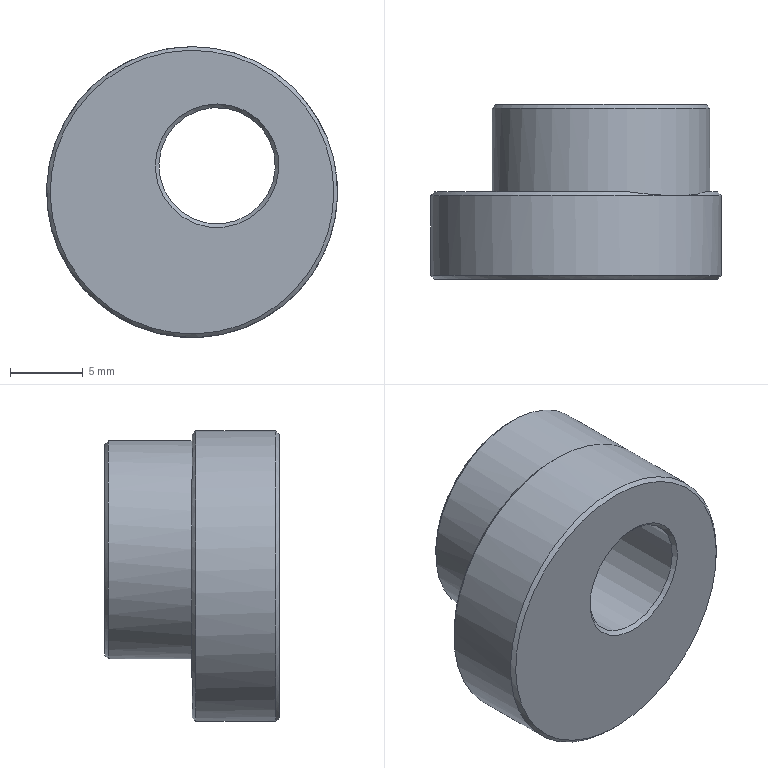Component | NX | ECCENTRIC_WHEEL | 1 solid | 11 faces | box 20 x 12 x 20 mm | volume 2335 mm3 | cone 5 | plane 3 | cylinder 3 | commonest cylinder face diameters 20 x1 15 x1 8 x1
STEP:
#1=CARTESIAN_POINT('',(0.,0.,0.));
#2=DIRECTION('',(0.,0.,1.));
#3=DIRECTION('',(1.,0.,0.));
#4=AXIS2_PLACEMENT_3D('',#1,#2,#3);
#5=CARTESIAN_POINT('',(7.185,-7.75,43.152));
#6=VERTEX_POINT('',#5);
#7=CARTESIAN_POINT('',(1.796,-7.75,48.282));
#8=VERTEX_POINT('',#7);
#9=CARTESIAN_POINT('',(-0.,-7.75,41.));
#10=DIRECTION('',(0.,1.,0.));
#11=DIRECTION('',(-0.7243,0.,0.6895));
#12=AXIS2_PLACEMENT_3D('',#9,#10,#11);
#13=CIRCLE('',#12,7.5);
#14=CARTESIAN_POINT('',(-1.724,-7.75,39.189));
#15=DIRECTION('',(0.,1.,0.));
#16=DIRECTION('',(-0.7243,0.,0.6895));
#17=AXIS2_PLACEMENT_3D('',#14,#15,#16);
#18=PLANE('',#17);
#19=CARTESIAN_POINT('',(0.,2.5));
#20=DIRECTION('',(1.,0.));
#21=AXIS2_PLACEMENT_2D('',#19,#20);
#22=CIRCLE('',#21,7.5);
#23=(GEOMETRIC_REPRESENTATION_CONTEXT(2)PARAMETRIC_REPRESENTATION_CONTEXT()REPRESENTATION_CONTEXT('',''));
#24=DEFINITIONAL_REPRESENTATION('',(#22),#23);
#25=PCURVE('',#18,#24);
#26=CARTESIAN_POINT('',(-0.,-1.75,41.));
#27=DIRECTION('',(0.,-1.,0.));
#28=DIRECTION('',(0.7243,0.,-0.6895));
#29=AXIS2_PLACEMENT_3D('',#26,#27,#28);
#30=CYLINDRICAL_SURFACE('',#29,7.5);
#31=CARTESIAN_POINT('',(9.425,6.));
#32=DIRECTION('',(-1.,0.));
#33=VECTOR('',#32,1.);
#34=LINE('',#31,#33);
#35=(GEOMETRIC_REPRESENTATION_CONTEXT(2)PARAMETRIC_REPRESENTATION_CONTEXT()REPRESENTATION_CONTEXT('',''));
#36=DEFINITIONAL_REPRESENTATION('',(#34),#35);
#37=PCURVE('',#30,#36);
#38=SURFACE_CURVE('',#13,(#25,#37),.PCURVE_S1.);
#39=EDGE_CURVE('',#6,#8,#38,.T.);
#40=ORIENTED_EDGE('',*,*,#39,.F.);
#41=CARTESIAN_POINT('',(-1.724,-7.75,39.189));
#42=DIRECTION('',(0.,1.,0.));
#43=DIRECTION('',(-0.7243,0.,0.6895));
#44=AXIS2_PLACEMENT_3D('',#41,#42,#43);
#45=CIRCLE('',#44,9.75);
#46=CARTESIAN_POINT('',(0.,0.));
#47=DIRECTION('',(1.,0.));
#48=AXIS2_PLACEMENT_2D('',#46,#47);
#49=CIRCLE('',#48,9.75);
#50=(GEOMETRIC_REPRESENTATION_CONTEXT(2)PARAMETRIC_REPRESENTATION_CONTEXT()REPRESENTATION_CONTEXT('',''));
#51=DEFINITIONAL_REPRESENTATION('',(#49),#50);
#52=PCURVE('',#18,#51);
#53=CARTESIAN_POINT('',(-1.724,-8.,39.189));
#54=DIRECTION('',(0.,-1.,0.));
#55=DIRECTION('',(0.7243,0.,-0.6895));
#56=AXIS2_PLACEMENT_3D('',#53,#54,#55);
#57=CONICAL_SURFACE('',#56,10.,0.7854);
#58=CARTESIAN_POINT('',(9.425,-0.25));
#59=DIRECTION('',(-1.,0.));
#60=VECTOR('',#59,1.);
#61=LINE('',#58,#60);
#62=(GEOMETRIC_REPRESENTATION_CONTEXT(2)PARAMETRIC_REPRESENTATION_CONTEXT()REPRESENTATION_CONTEXT('',''));
#63=DEFINITIONAL_REPRESENTATION('',(#61),#62);
#64=PCURVE('',#57,#63);
#65=SURFACE_CURVE('',#45,(#52,#64),.PCURVE_S1.);
#66=EDGE_CURVE('',#6,#8,#65,.T.);
#67=ORIENTED_EDGE('',*,*,#66,.T.);
#68=EDGE_LOOP('',(#40,#67));
#69=FACE_BOUND('',#68,.T.);
#70=ADVANCED_FACE('',(#69),#18,.T.);
#71=CARTESIAN_POINT('',(3.078,-13.75,38.07));
#72=VERTEX_POINT('',#71);
#73=CARTESIAN_POINT('',(-0.,-13.75,41.));
#74=DIRECTION('',(0.,1.,0.));
#75=DIRECTION('',(0.7243,0.,-0.6895));
#76=AXIS2_PLACEMENT_3D('',#73,#74,#75);
#77=CIRCLE('',#76,4.25);
#78=CARTESIAN_POINT('',(-1.724,-13.75,39.189));
#79=DIRECTION('',(0.,-1.,0.));
#80=DIRECTION('',(0.7243,0.,-0.6895));
#81=AXIS2_PLACEMENT_3D('',#78,#79,#80);
#82=PLANE('',#81);
#83=CARTESIAN_POINT('',(4.25,2.5));
#84=CARTESIAN_POINT('',(4.25,-4.861));
#85=CARTESIAN_POINT('',(-2.125,-1.181));
#86=CARTESIAN_POINT('',(-8.5,2.5));
#87=CARTESIAN_POINT('',(-2.125,6.181));
#88=CARTESIAN_POINT('',(4.25,9.861));
#89=CARTESIAN_POINT('',(4.25,2.5));
#90=(BOUNDED_CURVE()B_SPLINE_CURVE(2,(#83,#84,#85,#86,#87,#88,#89),.UNSPECIFIED.,.T.,.F.)B_SPLINE_CURVE_WITH_KNOTS((1,2,2,2,2,1),(-2.094,0.,2.094,4.189,6.283,8.378),.UNSPECIFIED.)CURVE()GEOMETRIC_REPRESENTATION_ITEM()RATIONAL_B_SPLINE_CURVE((1.,0.5,1.,0.5,1.,0.5,1.))REPRESENTATION_ITEM(''));
#91=(GEOMETRIC_REPRESENTATION_CONTEXT(2)PARAMETRIC_REPRESENTATION_CONTEXT()REPRESENTATION_CONTEXT('',''));
#92=DEFINITIONAL_REPRESENTATION('',(#90),#91);
#93=PCURVE('',#82,#92);
#94=CARTESIAN_POINT('',(-0.,-13.5,41.));
#95=DIRECTION('',(0.,-1.,0.));
#96=DIRECTION('',(0.7243,0.,-0.6895));
#97=AXIS2_PLACEMENT_3D('',#94,#95,#96);
#98=CONICAL_SURFACE('',#97,4.,0.7854);
#99=CARTESIAN_POINT('',(6.283,0.25));
#100=DIRECTION('',(-1.,-0.));
#101=VECTOR('',#100,1.);
#102=LINE('',#99,#101);
#103=(GEOMETRIC_REPRESENTATION_CONTEXT(2)PARAMETRIC_REPRESENTATION_CONTEXT()REPRESENTATION_CONTEXT('',''));
#104=DEFINITIONAL_REPRESENTATION('',(#102),#103);
#105=PCURVE('',#98,#104);
#106=SURFACE_CURVE('',#77,(#93,#105),.PCURVE_S1.);
#107=EDGE_CURVE('',#72,#72,#106,.T.);
#108=ORIENTED_EDGE('',*,*,#107,.T.);
#109=EDGE_LOOP('',(#108));
#110=FACE_BOUND('',#109,.T.);
#111=CARTESIAN_POINT('',(5.338,-13.75,32.467));
#112=VERTEX_POINT('',#111);
#113=CARTESIAN_POINT('',(-1.724,-13.75,39.189));
#114=DIRECTION('',(0.,-1.,0.));
#115=DIRECTION('',(0.7243,0.,-0.6895));
#116=AXIS2_PLACEMENT_3D('',#113,#114,#115);
#117=CIRCLE('',#116,9.75);
#118=CARTESIAN_POINT('',(0.,0.));
#119=DIRECTION('',(1.,0.));
#120=AXIS2_PLACEMENT_2D('',#118,#119);
#121=CIRCLE('',#120,9.75);
#122=(GEOMETRIC_REPRESENTATION_CONTEXT(2)PARAMETRIC_REPRESENTATION_CONTEXT()REPRESENTATION_CONTEXT('',''));
#123=DEFINITIONAL_REPRESENTATION('',(#121),#122);
#124=PCURVE('',#82,#123);
#125=CARTESIAN_POINT('',(-1.724,-13.5,39.189));
#126=DIRECTION('',(0.,1.,0.));
#127=DIRECTION('',(-0.7243,0.,0.6895));
#128=AXIS2_PLACEMENT_3D('',#125,#126,#127);
#129=CONICAL_SURFACE('',#128,10.,0.7854);
#130=CARTESIAN_POINT('',(9.425,-0.25));
#131=DIRECTION('',(-1.,0.));
#132=VECTOR('',#131,1.);
#133=LINE('',#130,#132);
#134=(GEOMETRIC_REPRESENTATION_CONTEXT(2)PARAMETRIC_REPRESENTATION_CONTEXT()REPRESENTATION_CONTEXT('',''));
#135=DEFINITIONAL_REPRESENTATION('',(#133),#134);
#136=PCURVE('',#129,#135);
#137=SURFACE_CURVE('',#117,(#124,#136),.PCURVE_S1.);
#138=EDGE_CURVE('',#112,#112,#137,.T.);
#139=ORIENTED_EDGE('',*,*,#138,.T.);
#140=EDGE_LOOP('',(#139));
#141=FACE_BOUND('',#140,.T.);
#142=ADVANCED_FACE('',(#110,#141),#82,.T.);
#143=CARTESIAN_POINT('',(5.519,-13.5,32.294));
#144=VERTEX_POINT('',#143);
#145=CARTESIAN_POINT('',(5.171,-13.5,46.432));
#146=VERTEX_POINT('',#145);
#147=CARTESIAN_POINT('',(-1.724,-13.5,39.189));
#148=DIRECTION('',(0.,1.,0.));
#149=DIRECTION('',(0.7243,0.,-0.6895));
#150=AXIS2_PLACEMENT_3D('',#147,#148,#149);
#151=CIRCLE('',#150,10.);
#152=CARTESIAN_POINT('',(-1.724,-13.75,39.189));
#153=DIRECTION('',(0.,1.,0.));
#154=DIRECTION('',(-0.7243,0.,0.6895));
#155=AXIS2_PLACEMENT_3D('',#152,#153,#154);
#156=CYLINDRICAL_SURFACE('',#155,10.);
#157=CARTESIAN_POINT('',(3.142,0.25));
#158=DIRECTION('',(1.,0.));
#159=VECTOR('',#158,1.);
#160=LINE('',#157,#159);
#161=(GEOMETRIC_REPRESENTATION_CONTEXT(2)PARAMETRIC_REPRESENTATION_CONTEXT()REPRESENTATION_CONTEXT('',''));
#162=DEFINITIONAL_REPRESENTATION('',(#160),#161);
#163=PCURVE('',#156,#162);
#164=CARTESIAN_POINT('',(3.142,0.));
#165=DIRECTION('',(1.,-0.));
#166=VECTOR('',#165,1.);
#167=LINE('',#164,#166);
#168=(GEOMETRIC_REPRESENTATION_CONTEXT(2)PARAMETRIC_REPRESENTATION_CONTEXT()REPRESENTATION_CONTEXT('',''));
#169=DEFINITIONAL_REPRESENTATION('',(#167),#168);
#170=PCURVE('',#129,#169);
#171=SURFACE_CURVE('',#151,(#163,#170),.PCURVE_S1.);
#172=EDGE_CURVE('',#144,#146,#171,.T.);
#173=ORIENTED_EDGE('',*,*,#172,.T.);
#174=CARTESIAN_POINT('',(5.171,-8.,46.432));
#175=VERTEX_POINT('',#174);
#176=CARTESIAN_POINT('',(5.171,-13.5,46.432));
#177=CARTESIAN_POINT('',(5.171,-8.,46.432));
#178=B_SPLINE_CURVE_WITH_KNOTS('',1,(#176,#177),.UNSPECIFIED.,.F.,.F.,(2,2),(0.25,5.75),.PIECEWISE_BEZIER_KNOTS.);
#179=CARTESIAN_POINT('',(7.854,0.));
#180=DIRECTION('',(0.,1.));
#181=VECTOR('',#180,1.);
#182=LINE('',#179,#181);
#183=(GEOMETRIC_REPRESENTATION_CONTEXT(2)PARAMETRIC_REPRESENTATION_CONTEXT()REPRESENTATION_CONTEXT('',''));
#184=DEFINITIONAL_REPRESENTATION('',(#182),#183);
#185=PCURVE('',#156,#184);
#186=CARTESIAN_POINT('',(1.571,0.));
#187=DIRECTION('',(0.,1.));
#188=VECTOR('',#187,1.);
#189=LINE('',#186,#188);
#190=(GEOMETRIC_REPRESENTATION_CONTEXT(2)PARAMETRIC_REPRESENTATION_CONTEXT()REPRESENTATION_CONTEXT('',''));
#191=DEFINITIONAL_REPRESENTATION('',(#189),#190);
#192=PCURVE('',#156,#191);
#193=SEAM_CURVE('',#178,(#185,#192),.PCURVE_S1.);
#194=EDGE_CURVE('',#146,#175,#193,.T.);
#195=ORIENTED_EDGE('',*,*,#194,.T.);
#196=CARTESIAN_POINT('',(-1.724,-8.,39.189));
#197=DIRECTION('',(0.,-1.,0.));
#198=DIRECTION('',(-0.7243,0.,0.6895));
#199=AXIS2_PLACEMENT_3D('',#196,#197,#198);
#200=CIRCLE('',#199,10.);
#201=CARTESIAN_POINT('',(12.566,5.75));
#202=DIRECTION('',(-1.,0.));
#203=VECTOR('',#202,1.);
#204=LINE('',#201,#203);
#205=(GEOMETRIC_REPRESENTATION_CONTEXT(2)PARAMETRIC_REPRESENTATION_CONTEXT()REPRESENTATION_CONTEXT('',''));
#206=DEFINITIONAL_REPRESENTATION('',(#204),#205);
#207=PCURVE('',#156,#206);
#208=CARTESIAN_POINT('',(-3.142,0.));
#209=DIRECTION('',(1.,0.));
#210=VECTOR('',#209,1.);
#211=LINE('',#208,#210);
#212=(GEOMETRIC_REPRESENTATION_CONTEXT(2)PARAMETRIC_REPRESENTATION_CONTEXT()REPRESENTATION_CONTEXT('',''));
#213=DEFINITIONAL_REPRESENTATION('',(#211),#212);
#214=PCURVE('',#57,#213);
#215=SURFACE_CURVE('',#200,(#207,#214),.PCURVE_S1.);
#216=EDGE_CURVE('',#175,#175,#215,.T.);
#217=ORIENTED_EDGE('',*,*,#216,.T.);
#218=ORIENTED_EDGE('',*,*,#194,.F.);
#219=CARTESIAN_POINT('',(-1.724,-13.5,39.189));
#220=DIRECTION('',(0.,1.,0.));
#221=DIRECTION('',(0.7243,0.,-0.6895));
#222=AXIS2_PLACEMENT_3D('',#219,#220,#221);
#223=CIRCLE('',#222,10.);
#224=CARTESIAN_POINT('',(-3.142,0.25));
#225=DIRECTION('',(1.,0.));
#226=VECTOR('',#225,1.);
#227=LINE('',#224,#226);
#228=(GEOMETRIC_REPRESENTATION_CONTEXT(2)PARAMETRIC_REPRESENTATION_CONTEXT()REPRESENTATION_CONTEXT('',''));
#229=DEFINITIONAL_REPRESENTATION('',(#227),#228);
#230=PCURVE('',#156,#229);
#231=CARTESIAN_POINT('',(3.142,-0.));
#232=DIRECTION('',(1.,0.));
#233=VECTOR('',#232,1.);
#234=LINE('',#231,#233);
#235=(GEOMETRIC_REPRESENTATION_CONTEXT(2)PARAMETRIC_REPRESENTATION_CONTEXT()REPRESENTATION_CONTEXT('',''));
#236=DEFINITIONAL_REPRESENTATION('',(#234),#235);
#237=PCURVE('',#129,#236);
#238=SURFACE_CURVE('',#223,(#230,#237),.PCURVE_S1.);
#239=EDGE_CURVE('',#146,#144,#238,.T.);
#240=ORIENTED_EDGE('',*,*,#239,.T.);
#241=EDGE_LOOP('',(#173,#195,#217,#218,#240));
#242=FACE_BOUND('',#241,.T.);
#243=ADVANCED_FACE('',(#242),#156,.T.);
#244=CARTESIAN_POINT('',(-5.432,-2.,46.171));
#245=VERTEX_POINT('',#244);
#246=CARTESIAN_POINT('',(7.185,-2.,43.152));
#247=VERTEX_POINT('',#246);
#248=CARTESIAN_POINT('',(-0.,-2.,41.));
#249=DIRECTION('',(0.,-1.,0.));
#250=DIRECTION('',(-0.7243,0.,0.6895));
#251=AXIS2_PLACEMENT_3D('',#248,#249,#250);
#252=CIRCLE('',#251,7.5);
#253=CARTESIAN_POINT('',(3.142,0.25));
#254=DIRECTION('',(1.,0.));
#255=VECTOR('',#254,1.);
#256=LINE('',#253,#255);
#257=(GEOMETRIC_REPRESENTATION_CONTEXT(2)PARAMETRIC_REPRESENTATION_CONTEXT()REPRESENTATION_CONTEXT('',''));
#258=DEFINITIONAL_REPRESENTATION('',(#256),#257);
#259=PCURVE('',#30,#258);
#260=CARTESIAN_POINT('',(-0.,-1.75,41.));
#261=DIRECTION('',(0.,-1.,0.));
#262=DIRECTION('',(0.7243,0.,-0.6895));
#263=AXIS2_PLACEMENT_3D('',#260,#261,#262);
#264=CONICAL_SURFACE('',#263,7.25,0.7854);
#265=CARTESIAN_POINT('',(3.142,0.25));
#266=DIRECTION('',(1.,-0.));
#267=VECTOR('',#266,1.);
#268=LINE('',#265,#267);
#269=(GEOMETRIC_REPRESENTATION_CONTEXT(2)PARAMETRIC_REPRESENTATION_CONTEXT()REPRESENTATION_CONTEXT('',''));
#270=DEFINITIONAL_REPRESENTATION('',(#268),#269);
#271=PCURVE('',#264,#270);
#272=SURFACE_CURVE('',#252,(#259,#271),.PCURVE_S1.);
#273=EDGE_CURVE('',#245,#247,#272,.T.);
#274=ORIENTED_EDGE('',*,*,#273,.T.);
#275=CARTESIAN_POINT('',(7.185,-2.,43.152));
#276=CARTESIAN_POINT('',(7.185,-7.75,43.152));
#277=B_SPLINE_CURVE_WITH_KNOTS('',1,(#275,#276),.UNSPECIFIED.,.F.,.F.,(2,2),(0.25,6.),.PIECEWISE_BEZIER_KNOTS.);
#278=CARTESIAN_POINT('',(7.335,0.));
#279=DIRECTION('',(0.,1.));
#280=VECTOR('',#279,1.);
#281=LINE('',#278,#280);
#282=(GEOMETRIC_REPRESENTATION_CONTEXT(2)PARAMETRIC_REPRESENTATION_CONTEXT()REPRESENTATION_CONTEXT('',''));
#283=DEFINITIONAL_REPRESENTATION('',(#281),#282);
#284=PCURVE('',#30,#283);
#285=CARTESIAN_POINT('',(1.052,0.));
#286=DIRECTION('',(0.,1.));
#287=VECTOR('',#286,1.);
#288=LINE('',#285,#287);
#289=(GEOMETRIC_REPRESENTATION_CONTEXT(2)PARAMETRIC_REPRESENTATION_CONTEXT()REPRESENTATION_CONTEXT('',''));
#290=DEFINITIONAL_REPRESENTATION('',(#288),#289);
#291=PCURVE('',#30,#290);
#292=SEAM_CURVE('',#277,(#284,#291),.PCURVE_S1.);
#293=EDGE_CURVE('',#247,#6,#292,.T.);
#294=ORIENTED_EDGE('',*,*,#293,.T.);
#295=ORIENTED_EDGE('',*,*,#39,.T.);
#296=CARTESIAN_POINT('',(1.796,-7.75,48.282));
#297=CARTESIAN_POINT('',(3.062,-7.916,47.969));
#298=CARTESIAN_POINT('',(4.219,-8.,47.339));
#299=CARTESIAN_POINT('',(5.171,-8.,46.432));
#300=B_SPLINE_CURVE_WITH_KNOTS('',3,(#296,#297,#298,#299),.UNSPECIFIED.,.F.,.F.,(4,4),(0.,1.),.PIECEWISE_BEZIER_KNOTS.);
#301=CARTESIAN_POINT('',(2.09,6.));
#302=CARTESIAN_POINT('',(2.082,6.008));
#303=CARTESIAN_POINT('',(2.066,6.022));
#304=CARTESIAN_POINT('',(2.042,6.043));
#305=CARTESIAN_POINT('',(2.019,6.063));
#306=CARTESIAN_POINT('',(1.995,6.083));
#307=CARTESIAN_POINT('',(1.972,6.101));
#308=CARTESIAN_POINT('',(1.948,6.118));
#309=CARTESIAN_POINT('',(1.925,6.134));
#310=CARTESIAN_POINT('',(1.901,6.149));
#311=CARTESIAN_POINT('',(1.878,6.163));
#312=CARTESIAN_POINT('',(1.854,6.175));
#313=CARTESIAN_POINT('',(1.831,6.187));
#314=CARTESIAN_POINT('',(1.807,6.198));
#315=CARTESIAN_POINT('',(1.784,6.208));
#316=CARTESIAN_POINT('',(1.76,6.217));
#317=CARTESIAN_POINT('',(1.737,6.225));
#318=CARTESIAN_POINT('',(1.713,6.231));
#319=CARTESIAN_POINT('',(1.69,6.237));
#320=CARTESIAN_POINT('',(1.666,6.242));
#321=CARTESIAN_POINT('',(1.642,6.245));
#322=CARTESIAN_POINT('',(1.618,6.248));
#323=CARTESIAN_POINT('',(1.595,6.25));
#324=CARTESIAN_POINT('',(1.579,6.25));
#325=CARTESIAN_POINT('',(1.571,6.25));
#326=B_SPLINE_CURVE_WITH_KNOTS('',3,(#301,#302,#303,#304,#305,#306,#307,#308,#309,#310,#311,#312,#313,#314,#315,#316,#317,#318,#319,#320,#321,#322,#323,#324,#325),.UNSPECIFIED.,.F.,.F.,(4,1,1,1,1,1,1,1,1,1,1,1,1,1,1,1,1,1,1,1,1,1,4),(0.,0.04545,0.09091,0.1364,0.1818,0.2273,0.2727,0.3182,0.3636,0.4091,0.4545,0.5,0.5455,0.5909,0.6364,0.6818,0.7273,0.7727,0.8182,0.8636,0.9091,0.9545,1.),.QUASI_UNIFORM_KNOTS.);
#327=(GEOMETRIC_REPRESENTATION_CONTEXT(2)PARAMETRIC_REPRESENTATION_CONTEXT()REPRESENTATION_CONTEXT('',''));
#328=DEFINITIONAL_REPRESENTATION('',(#326),#327);
#329=PCURVE('',#30,#328);
#330=CARTESIAN_POINT('',(1.962,-0.25));
#331=CARTESIAN_POINT('',(1.956,-0.2425));
#332=CARTESIAN_POINT('',(1.944,-0.2277));
#333=CARTESIAN_POINT('',(1.926,-0.2066));
#334=CARTESIAN_POINT('',(1.908,-0.1865));
#335=CARTESIAN_POINT('',(1.89,-0.1674));
#336=CARTESIAN_POINT('',(1.873,-0.1493));
#337=CARTESIAN_POINT('',(1.855,-0.1323));
#338=CARTESIAN_POINT('',(1.837,-0.1162));
#339=CARTESIAN_POINT('',(1.819,-0.1012));
#340=CARTESIAN_POINT('',(1.801,-0.08726));
#341=CARTESIAN_POINT('',(1.784,-0.07431));
#342=CARTESIAN_POINT('',(1.766,-0.0624));
#343=CARTESIAN_POINT('',(1.748,-0.05153));
#344=CARTESIAN_POINT('',(1.731,-0.04169));
#345=CARTESIAN_POINT('',(1.713,-0.03289));
#346=CARTESIAN_POINT('',(1.695,-0.02513));
#347=CARTESIAN_POINT('',(1.678,-0.0184));
#348=CARTESIAN_POINT('',(1.66,-0.01272));
#349=CARTESIAN_POINT('',(1.642,-0.008072));
#350=CARTESIAN_POINT('',(1.624,-0.004462));
#351=CARTESIAN_POINT('',(1.607,-0.001886));
#352=CARTESIAN_POINT('',(1.589,-0.0003423));
#353=CARTESIAN_POINT('',(1.577,0.00000004));
#354=CARTESIAN_POINT('',(1.571,0.));
#355=B_SPLINE_CURVE_WITH_KNOTS('',3,(#330,#331,#332,#333,#334,#335,#336,#337,#338,#339,#340,#341,#342,#343,#344,#345,#346,#347,#348,#349,#350,#351,#352,#353,#354),.UNSPECIFIED.,.F.,.F.,(4,1,1,1,1,1,1,1,1,1,1,1,1,1,1,1,1,1,1,1,1,1,4),(0.,0.04545,0.09091,0.1364,0.1818,0.2273,0.2727,0.3182,0.3636,0.4091,0.4545,0.5,0.5455,0.5909,0.6364,0.6818,0.7273,0.7727,0.8182,0.8636,0.9091,0.9545,1.),.QUASI_UNIFORM_KNOTS.);
#356=(GEOMETRIC_REPRESENTATION_CONTEXT(2)PARAMETRIC_REPRESENTATION_CONTEXT()REPRESENTATION_CONTEXT('',''));
#357=DEFINITIONAL_REPRESENTATION('',(#355),#356);
#358=PCURVE('',#57,#357);
#359=SURFACE_CURVE('',#300,(#329,#358),.PCURVE_S1.);
#360=EDGE_CURVE('',#8,#175,#359,.T.);
#361=ORIENTED_EDGE('',*,*,#360,.T.);
#362=CARTESIAN_POINT('',(5.171,-8.,46.432));
#363=CARTESIAN_POINT('',(6.12,-8.,45.529));
#364=CARTESIAN_POINT('',(6.812,-7.915,44.397));
#365=CARTESIAN_POINT('',(7.185,-7.75,43.152));
#366=B_SPLINE_CURVE_WITH_KNOTS('',3,(#362,#363,#364,#365),.UNSPECIFIED.,.F.,.F.,(4,4),(0.,1.),.PIECEWISE_BEZIER_KNOTS.);
#367=CARTESIAN_POINT('',(1.571,6.25));
#368=CARTESIAN_POINT('',(1.563,6.25));
#369=CARTESIAN_POINT('',(1.547,6.25));
#370=CARTESIAN_POINT('',(1.523,6.248));
#371=CARTESIAN_POINT('',(1.5,6.245));
#372=CARTESIAN_POINT('',(1.476,6.242));
#373=CARTESIAN_POINT('',(1.452,6.237));
#374=CARTESIAN_POINT('',(1.429,6.231));
#375=CARTESIAN_POINT('',(1.405,6.225));
#376=CARTESIAN_POINT('',(1.381,6.217));
#377=CARTESIAN_POINT('',(1.358,6.208));
#378=CARTESIAN_POINT('',(1.334,6.198));
#379=CARTESIAN_POINT('',(1.311,6.187));
#380=CARTESIAN_POINT('',(1.287,6.175));
#381=CARTESIAN_POINT('',(1.264,6.162));
#382=CARTESIAN_POINT('',(1.24,6.148));
#383=CARTESIAN_POINT('',(1.217,6.133));
#384=CARTESIAN_POINT('',(1.193,6.117));
#385=CARTESIAN_POINT('',(1.17,6.1));
#386=CARTESIAN_POINT('',(1.146,6.082));
#387=CARTESIAN_POINT('',(1.123,6.063));
#388=CARTESIAN_POINT('',(1.099,6.043));
#389=CARTESIAN_POINT('',(1.075,6.022));
#390=CARTESIAN_POINT('',(1.06,6.008));
#391=CARTESIAN_POINT('',(1.052,6.));
#392=B_SPLINE_CURVE_WITH_KNOTS('',3,(#367,#368,#369,#370,#371,#372,#373,#374,#375,#376,#377,#378,#379,#380,#381,#382,#383,#384,#385,#386,#387,#388,#389,#390,#391),.UNSPECIFIED.,.F.,.F.,(4,1,1,1,1,1,1,1,1,1,1,1,1,1,1,1,1,1,1,1,1,1,4),(0.,0.04545,0.09091,0.1364,0.1818,0.2273,0.2727,0.3182,0.3636,0.4091,0.4545,0.5,0.5455,0.5909,0.6364,0.6818,0.7273,0.7727,0.8182,0.8636,0.9091,0.9545,1.),.QUASI_UNIFORM_KNOTS.);
#393=(GEOMETRIC_REPRESENTATION_CONTEXT(2)PARAMETRIC_REPRESENTATION_CONTEXT()REPRESENTATION_CONTEXT('',''));
#394=DEFINITIONAL_REPRESENTATION('',(#392),#393);
#395=PCURVE('',#30,#394);
#396=CARTESIAN_POINT('',(7.854,0.));
#397=CARTESIAN_POINT('',(7.848,0.00000001));
#398=CARTESIAN_POINT('',(7.836,-0.000351));
#399=CARTESIAN_POINT('',(7.818,-0.001928));
#400=CARTESIAN_POINT('',(7.801,-0.004552));
#401=CARTESIAN_POINT('',(7.783,-0.008221));
#402=CARTESIAN_POINT('',(7.765,-0.01293));
#403=CARTESIAN_POINT('',(7.747,-0.01868));
#404=CARTESIAN_POINT('',(7.73,-0.02546));
#405=CARTESIAN_POINT('',(7.712,-0.03328));
#406=CARTESIAN_POINT('',(7.694,-0.04213));
#407=CARTESIAN_POINT('',(7.676,-0.052));
#408=CARTESIAN_POINT('',(7.659,-0.0629));
#409=CARTESIAN_POINT('',(7.641,-0.07482));
#410=CARTESIAN_POINT('',(7.623,-0.08777));
#411=CARTESIAN_POINT('',(7.606,-0.1017));
#412=CARTESIAN_POINT('',(7.588,-0.1167));
#413=CARTESIAN_POINT('',(7.57,-0.1327));
#414=CARTESIAN_POINT('',(7.552,-0.1497));
#415=CARTESIAN_POINT('',(7.534,-0.1677));
#416=CARTESIAN_POINT('',(7.516,-0.1867));
#417=CARTESIAN_POINT('',(7.499,-0.2068));
#418=CARTESIAN_POINT('',(7.481,-0.2278));
#419=CARTESIAN_POINT('',(7.469,-0.2425));
#420=CARTESIAN_POINT('',(7.463,-0.25));
#421=B_SPLINE_CURVE_WITH_KNOTS('',3,(#396,#397,#398,#399,#400,#401,#402,#403,#404,#405,#406,#407,#408,#409,#410,#411,#412,#413,#414,#415,#416,#417,#418,#419,#420),.UNSPECIFIED.,.F.,.F.,(4,1,1,1,1,1,1,1,1,1,1,1,1,1,1,1,1,1,1,1,1,1,4),(0.,0.04545,0.09091,0.1364,0.1818,0.2273,0.2727,0.3182,0.3636,0.4091,0.4545,0.5,0.5455,0.5909,0.6364,0.6818,0.7273,0.7727,0.8182,0.8636,0.9091,0.9545,1.),.QUASI_UNIFORM_KNOTS.);
#422=(GEOMETRIC_REPRESENTATION_CONTEXT(2)PARAMETRIC_REPRESENTATION_CONTEXT()REPRESENTATION_CONTEXT('',''));
#423=DEFINITIONAL_REPRESENTATION('',(#421),#422);
#424=PCURVE('',#57,#423);
#425=SURFACE_CURVE('',#366,(#395,#424),.PCURVE_S1.);
#426=EDGE_CURVE('',#175,#6,#425,.T.);
#427=ORIENTED_EDGE('',*,*,#426,.T.);
#428=ORIENTED_EDGE('',*,*,#293,.F.);
#429=CARTESIAN_POINT('',(-0.,-2.,41.));
#430=DIRECTION('',(0.,-1.,0.));
#431=DIRECTION('',(-0.7243,0.,0.6895));
#432=AXIS2_PLACEMENT_3D('',#429,#430,#431);
#433=CIRCLE('',#432,7.5);
#434=CARTESIAN_POINT('',(-3.142,0.25));
#435=DIRECTION('',(1.,0.));
#436=VECTOR('',#435,1.);
#437=LINE('',#434,#436);
#438=(GEOMETRIC_REPRESENTATION_CONTEXT(2)PARAMETRIC_REPRESENTATION_CONTEXT()REPRESENTATION_CONTEXT('',''));
#439=DEFINITIONAL_REPRESENTATION('',(#437),#438);
#440=PCURVE('',#30,#439);
#441=CARTESIAN_POINT('',(3.142,0.25));
#442=DIRECTION('',(1.,0.));
#443=VECTOR('',#442,1.);
#444=LINE('',#441,#443);
#445=(GEOMETRIC_REPRESENTATION_CONTEXT(2)PARAMETRIC_REPRESENTATION_CONTEXT()REPRESENTATION_CONTEXT('',''));
#446=DEFINITIONAL_REPRESENTATION('',(#444),#445);
#447=PCURVE('',#264,#446);
#448=SURFACE_CURVE('',#433,(#440,#447),.PCURVE_S1.);
#449=EDGE_CURVE('',#247,#245,#448,.T.);
#450=ORIENTED_EDGE('',*,*,#449,.T.);
#451=EDGE_LOOP('',(#274,#294,#295,#361,#427,#428,#450));
#452=FACE_BOUND('',#451,.T.);
#453=ADVANCED_FACE('',(#452),#30,.T.);
#454=CARTESIAN_POINT('',(-3.078,-1.75,43.93));
#455=VERTEX_POINT('',#454);
#456=CARTESIAN_POINT('',(-0.,-1.75,41.));
#457=DIRECTION('',(0.,-1.,0.));
#458=DIRECTION('',(-0.7243,0.,0.6895));
#459=AXIS2_PLACEMENT_3D('',#456,#457,#458);
#460=CIRCLE('',#459,4.25);
#461=CARTESIAN_POINT('',(-0.,-1.75,41.));
#462=DIRECTION('',(0.,1.,0.));
#463=DIRECTION('',(-0.7243,0.,0.6895));
#464=AXIS2_PLACEMENT_3D('',#461,#462,#463);
#465=PLANE('',#464);
#466=CARTESIAN_POINT('',(4.25,0.));
#467=CARTESIAN_POINT('',(4.25,-7.361));
#468=CARTESIAN_POINT('',(-2.125,-3.681));
#469=CARTESIAN_POINT('',(-8.5,-0.));
#470=CARTESIAN_POINT('',(-2.125,3.681));
#471=CARTESIAN_POINT('',(4.25,7.361));
#472=CARTESIAN_POINT('',(4.25,0.));
#473=(BOUNDED_CURVE()B_SPLINE_CURVE(2,(#466,#467,#468,#469,#470,#471,#472),.UNSPECIFIED.,.T.,.F.)B_SPLINE_CURVE_WITH_KNOTS((1,2,2,2,2,1),(-2.094,0.,2.094,4.189,6.283,8.378),.UNSPECIFIED.)CURVE()GEOMETRIC_REPRESENTATION_ITEM()RATIONAL_B_SPLINE_CURVE((1.,0.5,1.,0.5,1.,0.5,1.))REPRESENTATION_ITEM(''));
#474=(GEOMETRIC_REPRESENTATION_CONTEXT(2)PARAMETRIC_REPRESENTATION_CONTEXT()REPRESENTATION_CONTEXT('',''));
#475=DEFINITIONAL_REPRESENTATION('',(#473),#474);
#476=PCURVE('',#465,#475);
#477=CARTESIAN_POINT('',(-0.,-2.,41.));
#478=DIRECTION('',(0.,1.,0.));
#479=DIRECTION('',(-0.7243,0.,0.6895));
#480=AXIS2_PLACEMENT_3D('',#477,#478,#479);
#481=CONICAL_SURFACE('',#480,4.,0.7854);
#482=CARTESIAN_POINT('',(6.283,0.25));
#483=DIRECTION('',(-1.,0.));
#484=VECTOR('',#483,1.);
#485=LINE('',#482,#484);
#486=(GEOMETRIC_REPRESENTATION_CONTEXT(2)PARAMETRIC_REPRESENTATION_CONTEXT()REPRESENTATION_CONTEXT('',''));
#487=DEFINITIONAL_REPRESENTATION('',(#485),#486);
#488=PCURVE('',#481,#487);
#489=SURFACE_CURVE('',#460,(#476,#488),.PCURVE_S1.);
#490=EDGE_CURVE('',#455,#455,#489,.T.);
#491=ORIENTED_EDGE('',*,*,#490,.T.);
#492=EDGE_LOOP('',(#491));
#493=FACE_BOUND('',#492,.T.);
#494=CARTESIAN_POINT('',(-5.251,-1.75,45.999));
#495=VERTEX_POINT('',#494);
#496=CARTESIAN_POINT('',(-0.,-1.75,41.));
#497=DIRECTION('',(0.,1.,0.));
#498=DIRECTION('',(-0.7243,0.,0.6895));
#499=AXIS2_PLACEMENT_3D('',#496,#497,#498);
#500=CIRCLE('',#499,7.25);
#501=CARTESIAN_POINT('',(0.,0.));
#502=DIRECTION('',(1.,0.));
#503=AXIS2_PLACEMENT_2D('',#501,#502);
#504=CIRCLE('',#503,7.25);
#505=(GEOMETRIC_REPRESENTATION_CONTEXT(2)PARAMETRIC_REPRESENTATION_CONTEXT()REPRESENTATION_CONTEXT('',''));
#506=DEFINITIONAL_REPRESENTATION('',(#504),#505);
#507=PCURVE('',#465,#506);
#508=CARTESIAN_POINT('',(9.425,0.));
#509=DIRECTION('',(-1.,0.));
#510=VECTOR('',#509,1.);
#511=LINE('',#508,#510);
#512=(GEOMETRIC_REPRESENTATION_CONTEXT(2)PARAMETRIC_REPRESENTATION_CONTEXT()REPRESENTATION_CONTEXT('',''));
#513=DEFINITIONAL_REPRESENTATION('',(#511),#512);
#514=PCURVE('',#264,#513);
#515=SURFACE_CURVE('',#500,(#507,#514),.PCURVE_S1.);
#516=EDGE_CURVE('',#495,#495,#515,.T.);
#517=ORIENTED_EDGE('',*,*,#516,.T.);
#518=EDGE_LOOP('',(#517));
#519=FACE_BOUND('',#518,.T.);
#520=ADVANCED_FACE('',(#493,#519),#465,.T.);
#521=CARTESIAN_POINT('',(-2.897,-13.5,43.758));
#522=VERTEX_POINT('',#521);
#523=CARTESIAN_POINT('',(2.897,-13.5,38.242));
#524=VERTEX_POINT('',#523);
#525=CARTESIAN_POINT('',(-0.,-13.5,41.));
#526=DIRECTION('',(0.,-1.,0.));
#527=DIRECTION('',(0.7243,0.,-0.6895));
#528=AXIS2_PLACEMENT_3D('',#525,#526,#527);
#529=CIRCLE('',#528,4.);
#530=CARTESIAN_POINT('',(-0.,-19.55,41.));
#531=DIRECTION('',(0.,1.,0.));
#532=DIRECTION('',(-0.7243,0.,0.6895));
#533=AXIS2_PLACEMENT_3D('',#530,#531,#532);
#534=CYLINDRICAL_SURFACE('',#533,4.);
#535=CARTESIAN_POINT('',(9.425,6.05));
#536=DIRECTION('',(-1.,0.));
#537=VECTOR('',#536,1.);
#538=LINE('',#535,#537);
#539=(GEOMETRIC_REPRESENTATION_CONTEXT(2)PARAMETRIC_REPRESENTATION_CONTEXT()REPRESENTATION_CONTEXT('',''));
#540=DEFINITIONAL_REPRESENTATION('',(#538),#539);
#541=PCURVE('',#534,#540);
#542=CARTESIAN_POINT('',(0.,0.));
#543=DIRECTION('',(1.,-0.));
#544=VECTOR('',#543,1.);
#545=LINE('',#542,#544);
#546=(GEOMETRIC_REPRESENTATION_CONTEXT(2)PARAMETRIC_REPRESENTATION_CONTEXT()REPRESENTATION_CONTEXT('',''));
#547=DEFINITIONAL_REPRESENTATION('',(#545),#546);
#548=PCURVE('',#98,#547);
#549=SURFACE_CURVE('',#529,(#541,#548),.PCURVE_S1.);
#550=EDGE_CURVE('',#522,#524,#549,.T.);
#551=ORIENTED_EDGE('',*,*,#550,.F.);
#552=CARTESIAN_POINT('',(-2.897,-2.,43.758));
#553=VERTEX_POINT('',#552);
#554=CARTESIAN_POINT('',(-2.897,-13.5,43.758));
#555=CARTESIAN_POINT('',(-2.897,-2.,43.758));
#556=B_SPLINE_CURVE_WITH_KNOTS('',1,(#554,#555),.UNSPECIFIED.,.F.,.F.,(2,2),(6.05,17.55),.PIECEWISE_BEZIER_KNOTS.);
#557=CARTESIAN_POINT('',(6.283,0.));
#558=DIRECTION('',(0.,1.));
#559=VECTOR('',#558,1.);
#560=LINE('',#557,#559);
#561=(GEOMETRIC_REPRESENTATION_CONTEXT(2)PARAMETRIC_REPRESENTATION_CONTEXT()REPRESENTATION_CONTEXT('',''));
#562=DEFINITIONAL_REPRESENTATION('',(#560),#561);
#563=PCURVE('',#534,#562);
#564=CARTESIAN_POINT('',(0.,0.));
#565=DIRECTION('',(0.,1.));
#566=VECTOR('',#565,1.);
#567=LINE('',#564,#566);
#568=(GEOMETRIC_REPRESENTATION_CONTEXT(2)PARAMETRIC_REPRESENTATION_CONTEXT()REPRESENTATION_CONTEXT('',''));
#569=DEFINITIONAL_REPRESENTATION('',(#567),#568);
#570=PCURVE('',#534,#569);
#571=SEAM_CURVE('',#556,(#563,#570),.PCURVE_S1.);
#572=EDGE_CURVE('',#522,#553,#571,.T.);
#573=ORIENTED_EDGE('',*,*,#572,.T.);
#574=CARTESIAN_POINT('',(-0.,-2.,41.));
#575=DIRECTION('',(0.,1.,0.));
#576=DIRECTION('',(-0.7243,0.,0.6895));
#577=AXIS2_PLACEMENT_3D('',#574,#575,#576);
#578=CIRCLE('',#577,4.);
#579=CARTESIAN_POINT('',(0.,17.55));
#580=DIRECTION('',(1.,0.));
#581=VECTOR('',#580,1.);
#582=LINE('',#579,#581);
#583=(GEOMETRIC_REPRESENTATION_CONTEXT(2)PARAMETRIC_REPRESENTATION_CONTEXT()REPRESENTATION_CONTEXT('',''));
#584=DEFINITIONAL_REPRESENTATION('',(#582),#583);
#585=PCURVE('',#534,#584);
#586=CARTESIAN_POINT('',(0.,0.));
#587=DIRECTION('',(1.,0.));
#588=VECTOR('',#587,1.);
#589=LINE('',#586,#588);
#590=(GEOMETRIC_REPRESENTATION_CONTEXT(2)PARAMETRIC_REPRESENTATION_CONTEXT()REPRESENTATION_CONTEXT('',''));
#591=DEFINITIONAL_REPRESENTATION('',(#589),#590);
#592=PCURVE('',#481,#591);
#593=SURFACE_CURVE('',#578,(#585,#592),.PCURVE_S1.);
#594=EDGE_CURVE('',#553,#553,#593,.T.);
#595=ORIENTED_EDGE('',*,*,#594,.F.);
#596=ORIENTED_EDGE('',*,*,#572,.F.);
#597=CARTESIAN_POINT('',(-0.,-13.5,41.));
#598=DIRECTION('',(0.,-1.,0.));
#599=DIRECTION('',(0.7243,0.,-0.6895));
#600=AXIS2_PLACEMENT_3D('',#597,#598,#599);
#601=CIRCLE('',#600,4.);
#602=CARTESIAN_POINT('',(3.142,6.05));
#603=DIRECTION('',(-1.,0.));
#604=VECTOR('',#603,1.);
#605=LINE('',#602,#604);
#606=(GEOMETRIC_REPRESENTATION_CONTEXT(2)PARAMETRIC_REPRESENTATION_CONTEXT()REPRESENTATION_CONTEXT('',''));
#607=DEFINITIONAL_REPRESENTATION('',(#605),#606);
#608=PCURVE('',#534,#607);
#609=CARTESIAN_POINT('',(0.,-0.));
#610=DIRECTION('',(1.,0.));
#611=VECTOR('',#610,1.);
#612=LINE('',#609,#611);
#613=(GEOMETRIC_REPRESENTATION_CONTEXT(2)PARAMETRIC_REPRESENTATION_CONTEXT()REPRESENTATION_CONTEXT('',''));
#614=DEFINITIONAL_REPRESENTATION('',(#612),#613);
#615=PCURVE('',#98,#614);
#616=SURFACE_CURVE('',#601,(#608,#615),.PCURVE_S1.);
#617=EDGE_CURVE('',#524,#522,#616,.T.);
#618=ORIENTED_EDGE('',*,*,#617,.F.);
#619=EDGE_LOOP('',(#551,#573,#595,#596,#618));
#620=FACE_BOUND('',#619,.F.);
#621=ADVANCED_FACE('',(#620),#534,.F.);
#622=ORIENTED_EDGE('',*,*,#107,.T.);
#623=CARTESIAN_POINT('',(2.897,-13.5,38.242));
#624=CARTESIAN_POINT('',(3.078,-13.75,38.07));
#625=B_SPLINE_CURVE_WITH_KNOTS('',1,(#623,#624),.UNSPECIFIED.,.F.,.F.,(2,2),(-0.,0.3536),.PIECEWISE_BEZIER_KNOTS.);
#626=CARTESIAN_POINT('',(0.,0.));
#627=DIRECTION('',(0.,1.));
#628=VECTOR('',#627,1.);
#629=LINE('',#626,#628);
#630=(GEOMETRIC_REPRESENTATION_CONTEXT(2)PARAMETRIC_REPRESENTATION_CONTEXT()REPRESENTATION_CONTEXT('',''));
#631=DEFINITIONAL_REPRESENTATION('',(#629),#630);
#632=PCURVE('',#98,#631);
#633=CARTESIAN_POINT('',(6.283,0.));
#634=DIRECTION('',(0.,1.));
#635=VECTOR('',#634,1.);
#636=LINE('',#633,#635);
#637=(GEOMETRIC_REPRESENTATION_CONTEXT(2)PARAMETRIC_REPRESENTATION_CONTEXT()REPRESENTATION_CONTEXT('',''));
#638=DEFINITIONAL_REPRESENTATION('',(#636),#637);
#639=PCURVE('',#98,#638);
#640=SEAM_CURVE('',#625,(#632,#639),.PCURVE_S1.);
#641=EDGE_CURVE('',#524,#72,#640,.T.);
#642=ORIENTED_EDGE('',*,*,#641,.F.);
#643=ORIENTED_EDGE('',*,*,#617,.T.);
#644=ORIENTED_EDGE('',*,*,#550,.T.);
#645=ORIENTED_EDGE('',*,*,#641,.T.);
#646=EDGE_LOOP('',(#622,#642,#643,#644,#645));
#647=FACE_BOUND('',#646,.F.);
#648=ADVANCED_FACE('',(#647),#98,.F.);
#649=ORIENTED_EDGE('',*,*,#490,.T.);
#650=CARTESIAN_POINT('',(-2.897,-2.,43.758));
#651=CARTESIAN_POINT('',(-3.078,-1.75,43.93));
#652=B_SPLINE_CURVE_WITH_KNOTS('',1,(#650,#651),.UNSPECIFIED.,.F.,.F.,(2,2),(0.,0.3536),.PIECEWISE_BEZIER_KNOTS.);
#653=CARTESIAN_POINT('',(0.,0.));
#654=DIRECTION('',(0.,1.));
#655=VECTOR('',#654,1.);
#656=LINE('',#653,#655);
#657=(GEOMETRIC_REPRESENTATION_CONTEXT(2)PARAMETRIC_REPRESENTATION_CONTEXT()REPRESENTATION_CONTEXT('',''));
#658=DEFINITIONAL_REPRESENTATION('',(#656),#657);
#659=PCURVE('',#481,#658);
#660=CARTESIAN_POINT('',(6.283,0.));
#661=DIRECTION('',(0.,1.));
#662=VECTOR('',#661,1.);
#663=LINE('',#660,#662);
#664=(GEOMETRIC_REPRESENTATION_CONTEXT(2)PARAMETRIC_REPRESENTATION_CONTEXT()REPRESENTATION_CONTEXT('',''));
#665=DEFINITIONAL_REPRESENTATION('',(#663),#664);
#666=PCURVE('',#481,#665);
#667=SEAM_CURVE('',#652,(#659,#666),.PCURVE_S1.);
#668=EDGE_CURVE('',#553,#455,#667,.T.);
#669=ORIENTED_EDGE('',*,*,#668,.F.);
#670=ORIENTED_EDGE('',*,*,#594,.T.);
#671=ORIENTED_EDGE('',*,*,#668,.T.);
#672=EDGE_LOOP('',(#649,#669,#670,#671));
#673=FACE_BOUND('',#672,.F.);
#674=ADVANCED_FACE('',(#673),#481,.F.);
#675=ORIENTED_EDGE('',*,*,#138,.F.);
#676=CARTESIAN_POINT('',(5.338,-13.75,32.467));
#677=CARTESIAN_POINT('',(5.519,-13.5,32.294));
#678=B_SPLINE_CURVE_WITH_KNOTS('',1,(#676,#677),.UNSPECIFIED.,.F.,.F.,(2,2),(-0.3536,0.),.PIECEWISE_BEZIER_KNOTS.);
#679=CARTESIAN_POINT('',(9.425,0.));
#680=DIRECTION('',(0.,1.));
#681=VECTOR('',#680,1.);
#682=LINE('',#679,#681);
#683=(GEOMETRIC_REPRESENTATION_CONTEXT(2)PARAMETRIC_REPRESENTATION_CONTEXT()REPRESENTATION_CONTEXT('',''));
#684=DEFINITIONAL_REPRESENTATION('',(#682),#683);
#685=PCURVE('',#129,#684);
#686=CARTESIAN_POINT('',(3.142,0.));
#687=DIRECTION('',(0.,1.));
#688=VECTOR('',#687,1.);
#689=LINE('',#686,#688);
#690=(GEOMETRIC_REPRESENTATION_CONTEXT(2)PARAMETRIC_REPRESENTATION_CONTEXT()REPRESENTATION_CONTEXT('',''));
#691=DEFINITIONAL_REPRESENTATION('',(#689),#690);
#692=PCURVE('',#129,#691);
#693=SEAM_CURVE('',#678,(#685,#692),.PCURVE_S1.);
#694=EDGE_CURVE('',#112,#144,#693,.T.);
#695=ORIENTED_EDGE('',*,*,#694,.T.);
#696=ORIENTED_EDGE('',*,*,#239,.F.);
#697=ORIENTED_EDGE('',*,*,#172,.F.);
#698=ORIENTED_EDGE('',*,*,#694,.F.);
#699=EDGE_LOOP('',(#675,#695,#696,#697,#698));
#700=FACE_BOUND('',#699,.T.);
#701=ADVANCED_FACE('',(#700),#129,.T.);
#702=ORIENTED_EDGE('',*,*,#360,.F.);
#703=ORIENTED_EDGE('',*,*,#66,.F.);
#704=ORIENTED_EDGE('',*,*,#426,.F.);
#705=ORIENTED_EDGE('',*,*,#216,.F.);
#706=EDGE_LOOP('',(#702,#703,#704,#705));
#707=FACE_BOUND('',#706,.T.);
#708=ADVANCED_FACE('',(#707),#57,.T.);
#709=ORIENTED_EDGE('',*,*,#273,.F.);
#710=CARTESIAN_POINT('',(-5.251,-1.75,45.999));
#711=CARTESIAN_POINT('',(-5.432,-2.,46.171));
#712=B_SPLINE_CURVE_WITH_KNOTS('',1,(#710,#711),.UNSPECIFIED.,.F.,.F.,(2,2),(0.,0.3536),.PIECEWISE_BEZIER_KNOTS.);
#713=CARTESIAN_POINT('',(3.142,0.));
#714=DIRECTION('',(0.,1.));
#715=VECTOR('',#714,1.);
#716=LINE('',#713,#715);
#717=(GEOMETRIC_REPRESENTATION_CONTEXT(2)PARAMETRIC_REPRESENTATION_CONTEXT()REPRESENTATION_CONTEXT('',''));
#718=DEFINITIONAL_REPRESENTATION('',(#716),#717);
#719=PCURVE('',#264,#718);
#720=CARTESIAN_POINT('',(9.425,0.));
#721=DIRECTION('',(0.,1.));
#722=VECTOR('',#721,1.);
#723=LINE('',#720,#722);
#724=(GEOMETRIC_REPRESENTATION_CONTEXT(2)PARAMETRIC_REPRESENTATION_CONTEXT()REPRESENTATION_CONTEXT('',''));
#725=DEFINITIONAL_REPRESENTATION('',(#723),#724);
#726=PCURVE('',#264,#725);
#727=SEAM_CURVE('',#712,(#719,#726),.PCURVE_S1.);
#728=EDGE_CURVE('',#495,#245,#727,.T.);
#729=ORIENTED_EDGE('',*,*,#728,.F.);
#730=ORIENTED_EDGE('',*,*,#516,.F.);
#731=ORIENTED_EDGE('',*,*,#728,.T.);
#732=ORIENTED_EDGE('',*,*,#449,.F.);
#733=EDGE_LOOP('',(#709,#729,#730,#731,#732));
#734=FACE_BOUND('',#733,.T.);
#735=ADVANCED_FACE('',(#734),#264,.T.);
#736=CLOSED_SHELL('',(#70,#142,#243,#453,#520,#621,#648,#674,#701,#708,#735));
#737=MANIFOLD_SOLID_BREP('',#736);
#738=(LENGTH_UNIT()NAMED_UNIT(*)SI_UNIT(.MILLI.,.METRE.));
#739=UNCERTAINTY_MEASURE_WITH_UNIT(LENGTH_MEASURE(0.0001),#738,'','');
#740=(NAMED_UNIT(*)PLANE_ANGLE_UNIT()SI_UNIT($,.RADIAN.));
#741=(NAMED_UNIT(*)SI_UNIT($,.STERADIAN.)SOLID_ANGLE_UNIT());
#742=(GEOMETRIC_REPRESENTATION_CONTEXT(3)GLOBAL_UNCERTAINTY_ASSIGNED_CONTEXT((#739))GLOBAL_UNIT_ASSIGNED_CONTEXT((#738,#740,#741))REPRESENTATION_CONTEXT('',''));
#743=ADVANCED_BREP_SHAPE_REPRESENTATION('',(#4,#737),#742);